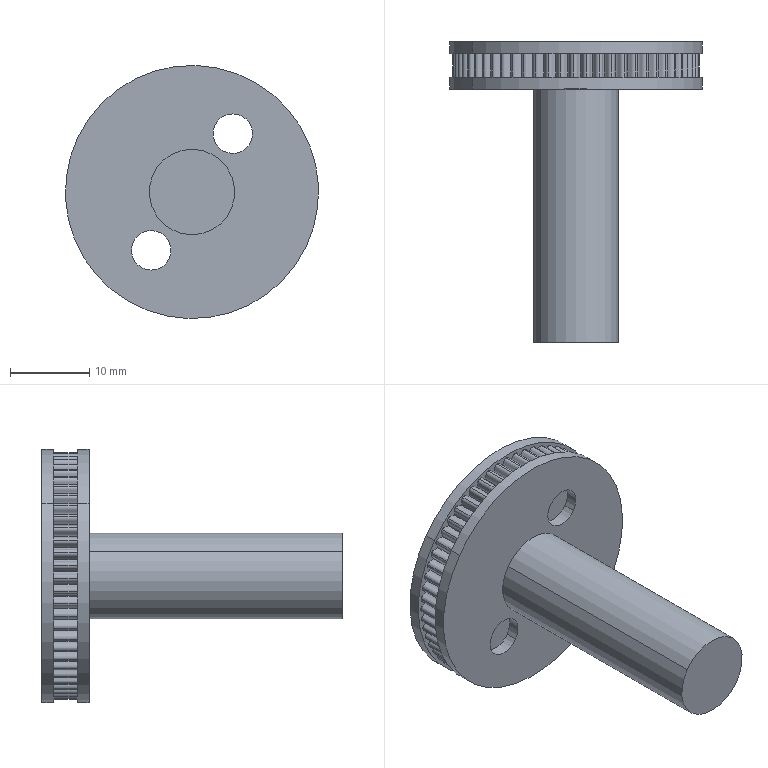Component | SolidWorks | BeltDrive-1 | 1 solid | 143 faces | box 32 x 38 x 32 mm | volume 5637 mm3 | spline 120 | cylinder 16 | plane 7 | commonest cylinder face diameters 5 x8 32 x4 10.8 x2 27.5 x2
build123d program:
from build123d import *

# Parameters (mm, degrees)
SKETCH1_R           = 16
SKETCH1_R_2         = 2.5
BOSS_EXTRUDE1_DEPTH = 1.5
SKETCH2_R           = 14.75
SKETCH2_R_2         = 13.75
BOSS_EXTRUDE2_DEPTH = 3
SKETCH3_R           = 16
SKETCH3_R_2         = 2.5
BOSS_EXTRUDE3_DEPTH = 1.5
SKETCH4_R           = 14.6
BOSS_EXTRUDE4_DEPTH = 3
SKETCH7_R           = 5.4
BOSS_EXTRUDE6_DEPTH = 32


with BuildPart() as part:
    # Sketch1 → Boss-Extrude1 (new body)
    with BuildSketch(Plane.XY):
        Circle(SKETCH1_R)
        with Locations((0, 9)):
            Circle(SKETCH1_R_2, mode=Mode.SUBTRACT)
        with Locations((0, -9)):
            Circle(SKETCH1_R_2, mode=Mode.SUBTRACT)
    extrude(amount=BOSS_EXTRUDE1_DEPTH)

    # Sketch2 → Boss-Extrude2 (add)
    with BuildSketch(Plane.XY.offset(1.5)):
        Circle(SKETCH2_R)
        Circle(SKETCH2_R_2, mode=Mode.SUBTRACT)
    extrude(amount=BOSS_EXTRUDE2_DEPTH)

    # Sketch3 → Boss-Extrude3 (add)
    with BuildSketch(Plane.XY.offset(4.5)):
        Circle(SKETCH3_R)
        with Locations((0, -9)):
            Circle(SKETCH3_R_2, mode=Mode.SUBTRACT)
        with Locations((0, 9)):
            Circle(SKETCH3_R_2, mode=Mode.SUBTRACT)
    extrude(amount=BOSS_EXTRUDE3_DEPTH)

    # Sketch4 → Boss-Extrude4 (add)
    with BuildSketch(Plane.XY.offset(1.5)):
        with BuildLine():
            add(Edge.make_bspline(
                [(0, 15.55), (-0.5399, 15.534), (-0.4124, 15.038), (-0.772, 14.73)],
                knots=[0, 0, 0, 0, 1, 1, 1, 1], degree=3))
            add(Edge.make_bspline(
                [(-1.625, 15.465), (-1.087, 15.505), (-1.162, 14.998), (-0.772, 14.73)],
                knots=[0, 0, 0, 0, 1, 1, 1, 1], degree=3))
            add(Edge.make_bspline(
                [(-1.625, 15.465), (-2.161, 15.392), (-1.982, 14.912), (-2.307, 14.568)],
                knots=[0, 0, 0, 0, 1, 1, 1, 1], degree=3))
            add(Edge.make_bspline(
                [(-3.233, 15.21), (-2.702, 15.307), (-2.723, 14.795), (-2.307, 14.568)],
                knots=[0, 0, 0, 0, 1, 1, 1, 1], degree=3))
            add(Edge.make_bspline(
                [(-3.233, 15.21), (-3.758, 15.082), (-3.53, 14.623), (-3.818, 14.247)],
                knots=[0, 0, 0, 0, 1, 1, 1, 1], degree=3))
            add(Edge.make_bspline(
                [(-4.805, 14.789), (-4.287, 14.94), (-4.255, 14.429), (-3.818, 14.247)],
                knots=[0, 0, 0, 0, 1, 1, 1, 1], degree=3))
            add(Edge.make_bspline(
                [(-4.805, 14.789), (-5.314, 14.607), (-5.039, 14.174), (-5.286, 13.77)],
                knots=[0, 0, 0, 0, 1, 1, 1, 1], degree=3))
            add(Edge.make_bspline(
                [(-6.325, 14.206), (-5.825, 14.41), (-5.74, 13.905), (-5.286, 13.77)],
                knots=[0, 0, 0, 0, 1, 1, 1, 1], degree=3))
            add(Edge.make_bspline(
                [(-6.325, 14.206), (-6.811, 13.971), (-6.493, 13.57), (-6.696, 13.142)],
                knots=[0, 0, 0, 0, 1, 1, 1, 1], degree=3))
            add(Edge.make_bspline(
                [(-7.775, 13.467), (-7.299, 13.723), (-7.162, 13.229), (-6.696, 13.142)],
                knots=[0, 0, 0, 0, 1, 1, 1, 1], degree=3))
            add(Edge.make_bspline(
                [(-7.775, 13.467), (-8.234, 13.183), (-7.876, 12.817), (-8.033, 12.37)],
                knots=[0, 0, 0, 0, 1, 1, 1, 1], degree=3))
            add(Edge.make_bspline(
                [(-9.14, 12.58), (-8.694, 12.884), (-8.505, 12.408), (-8.033, 12.37)],
                knots=[0, 0, 0, 0, 1, 1, 1, 1], degree=3))
            add(Edge.make_bspline(
                [(-9.14, 12.58), (-9.567, 12.25), (-9.173, 11.923), (-9.282, 11.463)],
                knots=[0, 0, 0, 0, 1, 1, 1, 1], degree=3))
            add(Edge.make_bspline(
                [(-10.405, 11.556), (-9.993, 11.905), (-9.756, 11.451), (-9.282, 11.463)],
                knots=[0, 0, 0, 0, 1, 1, 1, 1], degree=3))
            add(Edge.make_bspline(
                [(-10.405, 11.556), (-10.795, 11.183), (-10.369, 10.899), (-10.43, 10.43)],
                knots=[0, 0, 0, 0, 1, 1, 1, 1], degree=3))
            add(Edge.make_bspline(
                [(-11.556, 10.405), (-11.183, 10.795), (-10.899, 10.369), (-10.43, 10.43)],
                knots=[0, 0, 0, 0, 1, 1, 1, 1], degree=3))
            add(Edge.make_bspline(
                [(-11.556, 10.405), (-11.905, 9.993), (-11.451, 9.756), (-11.463, 9.282)],
                knots=[0, 0, 0, 0, 1, 1, 1, 1], degree=3))
            add(Edge.make_bspline(
                [(-12.58, 9.14), (-12.25, 9.567), (-11.923, 9.173), (-11.463, 9.282)],
                knots=[0, 0, 0, 0, 1, 1, 1, 1], degree=3))
            add(Edge.make_bspline(
                [(-12.58, 9.14), (-12.884, 8.694), (-12.408, 8.505), (-12.37, 8.033)],
                knots=[0, 0, 0, 0, 1, 1, 1, 1], degree=3))
            add(Edge.make_bspline(
                [(-13.467, 7.775), (-13.183, 8.234), (-12.817, 7.876), (-12.37, 8.033)],
                knots=[0, 0, 0, 0, 1, 1, 1, 1], degree=3))
            add(Edge.make_bspline(
                [(-13.467, 7.775), (-13.723, 7.299), (-13.229, 7.162), (-13.142, 6.696)],
                knots=[0, 0, 0, 0, 1, 1, 1, 1], degree=3))
            add(Edge.make_bspline(
                [(-14.206, 6.325), (-13.971, 6.811), (-13.57, 6.493), (-13.142, 6.696)],
                knots=[0, 0, 0, 0, 1, 1, 1, 1], degree=3))
            add(Edge.make_bspline(
                [(-14.206, 6.325), (-14.41, 5.825), (-13.905, 5.74), (-13.77, 5.286)],
                knots=[0, 0, 0, 0, 1, 1, 1, 1], degree=3))
            add(Edge.make_bspline(
                [(-14.789, 4.805), (-14.607, 5.314), (-14.174, 5.039), (-13.77, 5.286)],
                knots=[0, 0, 0, 0, 1, 1, 1, 1], degree=3))
            add(Edge.make_bspline(
                [(-14.789, 4.805), (-14.94, 4.287), (-14.429, 4.255), (-14.247, 3.818)],
                knots=[0, 0, 0, 0, 1, 1, 1, 1], degree=3))
            add(Edge.make_bspline(
                [(-15.21, 3.233), (-15.082, 3.758), (-14.623, 3.53), (-14.247, 3.818)],
                knots=[0, 0, 0, 0, 1, 1, 1, 1], degree=3))
            add(Edge.make_bspline(
                [(-15.21, 3.233), (-15.307, 2.702), (-14.795, 2.723), (-14.568, 2.307)],
                knots=[0, 0, 0, 0, 1, 1, 1, 1], degree=3))
            add(Edge.make_bspline(
                [(-15.465, 1.625), (-15.392, 2.161), (-14.912, 1.982), (-14.568, 2.307)],
                knots=[0, 0, 0, 0, 1, 1, 1, 1], degree=3))
            add(Edge.make_bspline(
                [(-15.465, 1.625), (-15.505, 1.087), (-14.998, 1.162), (-14.73, 0.772)],
                knots=[0, 0, 0, 0, 1, 1, 1, 1], degree=3))
            add(Edge.make_bspline(
                [(-15.55, 0), (-15.534, 0.5399), (-15.038, 0.4124), (-14.73, 0.772)],
                knots=[0, 0, 0, 0, 1, 1, 1, 1], degree=3))
            add(Edge.make_bspline(
                [(-15.55, 0), (-15.534, -0.5399), (-15.038, -0.4124), (-14.73, -0.772)],
                knots=[0, 0, 0, 0, 1, 1, 1, 1], degree=3))
            add(Edge.make_bspline(
                [(-15.465, -1.625), (-15.505, -1.087), (-14.998, -1.162), (-14.73, -0.772)],
                knots=[0, 0, 0, 0, 1, 1, 1, 1], degree=3))
            add(Edge.make_bspline(
                [(-15.465, -1.625), (-15.392, -2.161), (-14.912, -1.982), (-14.568, -2.307)],
                knots=[0, 0, 0, 0, 1, 1, 1, 1], degree=3))
            add(Edge.make_bspline(
                [(-15.21, -3.233), (-15.307, -2.702), (-14.795, -2.723), (-14.568, -2.307)],
                knots=[0, 0, 0, 0, 1, 1, 1, 1], degree=3))
            add(Edge.make_bspline(
                [(-15.21, -3.233), (-15.082, -3.758), (-14.623, -3.53), (-14.247, -3.818)],
                knots=[0, 0, 0, 0, 1, 1, 1, 1], degree=3))
            add(Edge.make_bspline(
                [(-14.789, -4.805), (-14.94, -4.287), (-14.429, -4.255), (-14.247, -3.818)],
                knots=[0, 0, 0, 0, 1, 1, 1, 1], degree=3))
            add(Edge.make_bspline(
                [(-14.789, -4.805), (-14.607, -5.314), (-14.174, -5.039), (-13.77, -5.286)],
                knots=[0, 0, 0, 0, 1, 1, 1, 1], degree=3))
            add(Edge.make_bspline(
                [(-14.206, -6.325), (-14.41, -5.825), (-13.905, -5.74), (-13.77, -5.286)],
                knots=[0, 0, 0, 0, 1, 1, 1, 1], degree=3))
            add(Edge.make_bspline(
                [(-14.206, -6.325), (-13.971, -6.811), (-13.57, -6.493), (-13.142, -6.696)],
                knots=[0, 0, 0, 0, 1, 1, 1, 1], degree=3))
            add(Edge.make_bspline(
                [(-13.467, -7.775), (-13.723, -7.299), (-13.229, -7.162), (-13.142, -6.696)],
                knots=[0, 0, 0, 0, 1, 1, 1, 1], degree=3))
            add(Edge.make_bspline(
                [(-13.467, -7.775), (-13.183, -8.234), (-12.817, -7.876), (-12.37, -8.033)],
                knots=[0, 0, 0, 0, 1, 1, 1, 1], degree=3))
            add(Edge.make_bspline(
                [(-12.58, -9.14), (-12.884, -8.694), (-12.408, -8.505), (-12.37, -8.033)],
                knots=[0, 0, 0, 0, 1, 1, 1, 1], degree=3))
            add(Edge.make_bspline(
                [(-12.58, -9.14), (-12.25, -9.567), (-11.923, -9.173), (-11.463, -9.282)],
                knots=[0, 0, 0, 0, 1, 1, 1, 1], degree=3))
            add(Edge.make_bspline(
                [(-11.556, -10.405), (-11.905, -9.993), (-11.451, -9.756), (-11.463, -9.282)],
                knots=[0, 0, 0, 0, 1, 1, 1, 1], degree=3))
            add(Edge.make_bspline(
                [(-11.556, -10.405), (-11.183, -10.795), (-10.899, -10.369), (-10.43, -10.43)],
                knots=[0, 0, 0, 0, 1, 1, 1, 1], degree=3))
            add(Edge.make_bspline(
                [(-10.405, -11.556), (-10.795, -11.183), (-10.369, -10.899), (-10.43, -10.43)],
                knots=[0, 0, 0, 0, 1, 1, 1, 1], degree=3))
            add(Edge.make_bspline(
                [(-10.405, -11.556), (-9.993, -11.905), (-9.756, -11.451), (-9.282, -11.463)],
                knots=[0, 0, 0, 0, 1, 1, 1, 1], degree=3))
            add(Edge.make_bspline(
                [(-9.14, -12.58), (-9.567, -12.25), (-9.173, -11.923), (-9.282, -11.463)],
                knots=[0, 0, 0, 0, 1, 1, 1, 1], degree=3))
            add(Edge.make_bspline(
                [(-9.14, -12.58), (-8.694, -12.884), (-8.505, -12.408), (-8.033, -12.37)],
                knots=[0, 0, 0, 0, 1, 1, 1, 1], degree=3))
            add(Edge.make_bspline(
                [(-7.775, -13.467), (-8.234, -13.183), (-7.876, -12.817), (-8.033, -12.37)],
                knots=[0, 0, 0, 0, 1, 1, 1, 1], degree=3))
            add(Edge.make_bspline(
                [(-7.775, -13.467), (-7.299, -13.723), (-7.162, -13.229), (-6.696, -13.142)],
                knots=[0, 0, 0, 0, 1, 1, 1, 1], degree=3))
            add(Edge.make_bspline(
                [(-6.325, -14.206), (-6.811, -13.971), (-6.493, -13.57), (-6.696, -13.142)],
                knots=[0, 0, 0, 0, 1, 1, 1, 1], degree=3))
            add(Edge.make_bspline(
                [(-6.325, -14.206), (-5.825, -14.41), (-5.74, -13.905), (-5.286, -13.77)],
                knots=[0, 0, 0, 0, 1, 1, 1, 1], degree=3))
            add(Edge.make_bspline(
                [(-4.805, -14.789), (-5.314, -14.607), (-5.039, -14.174), (-5.286, -13.77)],
                knots=[0, 0, 0, 0, 1, 1, 1, 1], degree=3))
            add(Edge.make_bspline(
                [(-4.805, -14.789), (-4.287, -14.94), (-4.255, -14.429), (-3.818, -14.247)],
                knots=[0, 0, 0, 0, 1, 1, 1, 1], degree=3))
            add(Edge.make_bspline(
                [(-3.233, -15.21), (-3.758, -15.082), (-3.53, -14.623), (-3.818, -14.247)],
                knots=[0, 0, 0, 0, 1, 1, 1, 1], degree=3))
            add(Edge.make_bspline(
                [(-3.233, -15.21), (-2.702, -15.307), (-2.723, -14.795), (-2.307, -14.568)],
                knots=[0, 0, 0, 0, 1, 1, 1, 1], degree=3))
            add(Edge.make_bspline(
                [(-1.625, -15.465), (-2.161, -15.392), (-1.982, -14.912), (-2.307, -14.568)],
                knots=[0, 0, 0, 0, 1, 1, 1, 1], degree=3))
            add(Edge.make_bspline(
                [(-1.625, -15.465), (-1.087, -15.505), (-1.162, -14.998), (-0.772, -14.73)],
                knots=[0, 0, 0, 0, 1, 1, 1, 1], degree=3))
            add(Edge.make_bspline(
                [(0, -15.55), (-0.5399, -15.534), (-0.4124, -15.038), (-0.772, -14.73)],
                knots=[0, 0, 0, 0, 1, 1, 1, 1], degree=3))
            add(Edge.make_bspline(
                [(0, -15.55), (0.5399, -15.534), (0.4124, -15.038), (0.772, -14.73)],
                knots=[0, 0, 0, 0, 1, 1, 1, 1], degree=3))
            add(Edge.make_bspline(
                [(1.625, -15.465), (1.087, -15.505), (1.162, -14.998), (0.772, -14.73)],
                knots=[0, 0, 0, 0, 1, 1, 1, 1], degree=3))
            add(Edge.make_bspline(
                [(1.625, -15.465), (2.161, -15.392), (1.982, -14.912), (2.307, -14.568)],
                knots=[0, 0, 0, 0, 1, 1, 1, 1], degree=3))
            add(Edge.make_bspline(
                [(3.233, -15.21), (2.702, -15.307), (2.723, -14.795), (2.307, -14.568)],
                knots=[0, 0, 0, 0, 1, 1, 1, 1], degree=3))
            add(Edge.make_bspline(
                [(3.233, -15.21), (3.758, -15.082), (3.53, -14.623), (3.818, -14.247)],
                knots=[0, 0, 0, 0, 1, 1, 1, 1], degree=3))
            add(Edge.make_bspline(
                [(4.805, -14.789), (4.287, -14.94), (4.255, -14.429), (3.818, -14.247)],
                knots=[0, 0, 0, 0, 1, 1, 1, 1], degree=3))
            add(Edge.make_bspline(
                [(4.805, -14.789), (5.314, -14.607), (5.039, -14.174), (5.286, -13.77)],
                knots=[0, 0, 0, 0, 1, 1, 1, 1], degree=3))
            add(Edge.make_bspline(
                [(6.325, -14.206), (5.825, -14.41), (5.74, -13.905), (5.286, -13.77)],
                knots=[0, 0, 0, 0, 1, 1, 1, 1], degree=3))
            add(Edge.make_bspline(
                [(6.325, -14.206), (6.811, -13.971), (6.493, -13.57), (6.696, -13.142)],
                knots=[0, 0, 0, 0, 1, 1, 1, 1], degree=3))
            add(Edge.make_bspline(
                [(7.775, -13.467), (7.299, -13.723), (7.162, -13.229), (6.696, -13.142)],
                knots=[0, 0, 0, 0, 1, 1, 1, 1], degree=3))
            add(Edge.make_bspline(
                [(7.775, -13.467), (8.234, -13.183), (7.876, -12.817), (8.033, -12.37)],
                knots=[0, 0, 0, 0, 1, 1, 1, 1], degree=3))
            add(Edge.make_bspline(
                [(9.14, -12.58), (8.694, -12.884), (8.505, -12.408), (8.033, -12.37)],
                knots=[0, 0, 0, 0, 1, 1, 1, 1], degree=3))
            add(Edge.make_bspline(
                [(9.14, -12.58), (9.567, -12.25), (9.173, -11.923), (9.282, -11.463)],
                knots=[0, 0, 0, 0, 1, 1, 1, 1], degree=3))
            add(Edge.make_bspline(
                [(10.405, -11.556), (9.993, -11.905), (9.756, -11.451), (9.282, -11.463)],
                knots=[0, 0, 0, 0, 1, 1, 1, 1], degree=3))
            add(Edge.make_bspline(
                [(10.405, -11.556), (10.795, -11.183), (10.369, -10.899), (10.43, -10.43)],
                knots=[0, 0, 0, 0, 1, 1, 1, 1], degree=3))
            add(Edge.make_bspline(
                [(11.556, -10.405), (11.183, -10.795), (10.899, -10.369), (10.43, -10.43)],
                knots=[0, 0, 0, 0, 1, 1, 1, 1], degree=3))
            add(Edge.make_bspline(
                [(11.556, -10.405), (11.905, -9.993), (11.451, -9.756), (11.463, -9.282)],
                knots=[0, 0, 0, 0, 1, 1, 1, 1], degree=3))
            add(Edge.make_bspline(
                [(12.58, -9.14), (12.25, -9.567), (11.923, -9.173), (11.463, -9.282)],
                knots=[0, 0, 0, 0, 1, 1, 1, 1], degree=3))
            add(Edge.make_bspline(
                [(12.58, -9.14), (12.884, -8.694), (12.408, -8.505), (12.37, -8.033)],
                knots=[0, 0, 0, 0, 1, 1, 1, 1], degree=3))
            add(Edge.make_bspline(
                [(13.467, -7.775), (13.183, -8.234), (12.817, -7.876), (12.37, -8.033)],
                knots=[0, 0, 0, 0, 1, 1, 1, 1], degree=3))
            add(Edge.make_bspline(
                [(13.467, -7.775), (13.723, -7.299), (13.229, -7.162), (13.142, -6.696)],
                knots=[0, 0, 0, 0, 1, 1, 1, 1], degree=3))
            add(Edge.make_bspline(
                [(14.206, -6.325), (13.971, -6.811), (13.57, -6.493), (13.142, -6.696)],
                knots=[0, 0, 0, 0, 1, 1, 1, 1], degree=3))
            add(Edge.make_bspline(
                [(14.206, -6.325), (14.41, -5.825), (13.905, -5.74), (13.77, -5.286)],
                knots=[0, 0, 0, 0, 1, 1, 1, 1], degree=3))
            add(Edge.make_bspline(
                [(14.789, -4.805), (14.607, -5.314), (14.174, -5.039), (13.77, -5.286)],
                knots=[0, 0, 0, 0, 1, 1, 1, 1], degree=3))
            add(Edge.make_bspline(
                [(14.789, -4.805), (14.94, -4.287), (14.429, -4.255), (14.247, -3.818)],
                knots=[0, 0, 0, 0, 1, 1, 1, 1], degree=3))
            add(Edge.make_bspline(
                [(15.21, -3.233), (15.082, -3.758), (14.623, -3.53), (14.247, -3.818)],
                knots=[0, 0, 0, 0, 1, 1, 1, 1], degree=3))
            add(Edge.make_bspline(
                [(15.21, -3.233), (15.307, -2.702), (14.795, -2.723), (14.568, -2.307)],
                knots=[0, 0, 0, 0, 1, 1, 1, 1], degree=3))
            add(Edge.make_bspline(
                [(15.465, -1.625), (15.392, -2.161), (14.912, -1.982), (14.568, -2.307)],
                knots=[0, 0, 0, 0, 1, 1, 1, 1], degree=3))
            add(Edge.make_bspline(
                [(15.465, -1.625), (15.505, -1.087), (14.998, -1.162), (14.73, -0.772)],
                knots=[0, 0, 0, 0, 1, 1, 1, 1], degree=3))
            add(Edge.make_bspline(
                [(15.55, 0), (15.534, -0.5399), (15.038, -0.4124), (14.73, -0.772)],
                knots=[0, 0, 0, 0, 1, 1, 1, 1], degree=3))
            add(Edge.make_bspline(
                [(15.55, 0), (15.534, 0.5399), (15.038, 0.4124), (14.73, 0.772)],
                knots=[0, 0, 0, 0, 1, 1, 1, 1], degree=3))
            add(Edge.make_bspline(
                [(15.465, 1.625), (15.505, 1.087), (14.998, 1.162), (14.73, 0.772)],
                knots=[0, 0, 0, 0, 1, 1, 1, 1], degree=3))
            add(Edge.make_bspline(
                [(15.465, 1.625), (15.392, 2.161), (14.912, 1.982), (14.568, 2.307)],
                knots=[0, 0, 0, 0, 1, 1, 1, 1], degree=3))
            add(Edge.make_bspline(
                [(15.21, 3.233), (15.307, 2.702), (14.795, 2.723), (14.568, 2.307)],
                knots=[0, 0, 0, 0, 1, 1, 1, 1], degree=3))
            add(Edge.make_bspline(
                [(15.21, 3.233), (15.082, 3.758), (14.623, 3.53), (14.247, 3.818)],
                knots=[0, 0, 0, 0, 1, 1, 1, 1], degree=3))
            add(Edge.make_bspline(
                [(14.789, 4.805), (14.94, 4.287), (14.429, 4.255), (14.247, 3.818)],
                knots=[0, 0, 0, 0, 1, 1, 1, 1], degree=3))
            add(Edge.make_bspline(
                [(14.789, 4.805), (14.607, 5.314), (14.174, 5.039), (13.77, 5.286)],
                knots=[0, 0, 0, 0, 1, 1, 1, 1], degree=3))
            add(Edge.make_bspline(
                [(14.206, 6.325), (14.41, 5.825), (13.905, 5.74), (13.77, 5.286)],
                knots=[0, 0, 0, 0, 1, 1, 1, 1], degree=3))
            add(Edge.make_bspline(
                [(14.206, 6.325), (13.971, 6.811), (13.57, 6.493), (13.142, 6.696)],
                knots=[0, 0, 0, 0, 1, 1, 1, 1], degree=3))
            add(Edge.make_bspline(
                [(13.467, 7.775), (13.723, 7.299), (13.229, 7.162), (13.142, 6.696)],
                knots=[0, 0, 0, 0, 1, 1, 1, 1], degree=3))
            add(Edge.make_bspline(
                [(13.467, 7.775), (13.183, 8.234), (12.817, 7.876), (12.37, 8.033)],
                knots=[0, 0, 0, 0, 1, 1, 1, 1], degree=3))
            add(Edge.make_bspline(
                [(12.58, 9.14), (12.884, 8.694), (12.408, 8.505), (12.37, 8.033)],
                knots=[0, 0, 0, 0, 1, 1, 1, 1], degree=3))
            add(Edge.make_bspline(
                [(12.58, 9.14), (12.25, 9.567), (11.923, 9.173), (11.463, 9.282)],
                knots=[0, 0, 0, 0, 1, 1, 1, 1], degree=3))
            add(Edge.make_bspline(
                [(11.556, 10.405), (11.905, 9.993), (11.451, 9.756), (11.463, 9.282)],
                knots=[0, 0, 0, 0, 1, 1, 1, 1], degree=3))
            add(Edge.make_bspline(
                [(11.556, 10.405), (11.183, 10.795), (10.899, 10.369), (10.43, 10.43)],
                knots=[0, 0, 0, 0, 1, 1, 1, 1], degree=3))
            add(Edge.make_bspline(
                [(10.405, 11.556), (10.795, 11.183), (10.369, 10.899), (10.43, 10.43)],
                knots=[0, 0, 0, 0, 1, 1, 1, 1], degree=3))
            add(Edge.make_bspline(
                [(10.405, 11.556), (9.993, 11.905), (9.756, 11.451), (9.282, 11.463)],
                knots=[0, 0, 0, 0, 1, 1, 1, 1], degree=3))
            add(Edge.make_bspline(
                [(9.14, 12.58), (9.567, 12.25), (9.173, 11.923), (9.282, 11.463)],
                knots=[0, 0, 0, 0, 1, 1, 1, 1], degree=3))
            add(Edge.make_bspline(
                [(9.14, 12.58), (8.694, 12.884), (8.505, 12.408), (8.033, 12.37)],
                knots=[0, 0, 0, 0, 1, 1, 1, 1], degree=3))
            add(Edge.make_bspline(
                [(7.775, 13.467), (8.234, 13.183), (7.876, 12.817), (8.033, 12.37)],
                knots=[0, 0, 0, 0, 1, 1, 1, 1], degree=3))
            add(Edge.make_bspline(
                [(7.775, 13.467), (7.299, 13.723), (7.162, 13.229), (6.696, 13.142)],
                knots=[0, 0, 0, 0, 1, 1, 1, 1], degree=3))
            add(Edge.make_bspline(
                [(6.325, 14.206), (6.811, 13.971), (6.493, 13.57), (6.696, 13.142)],
                knots=[0, 0, 0, 0, 1, 1, 1, 1], degree=3))
            add(Edge.make_bspline(
                [(6.325, 14.206), (5.825, 14.41), (5.74, 13.905), (5.286, 13.77)],
                knots=[0, 0, 0, 0, 1, 1, 1, 1], degree=3))
            add(Edge.make_bspline(
                [(4.805, 14.789), (5.314, 14.607), (5.039, 14.174), (5.286, 13.77)],
                knots=[0, 0, 0, 0, 1, 1, 1, 1], degree=3))
            add(Edge.make_bspline(
                [(4.805, 14.789), (4.287, 14.94), (4.255, 14.429), (3.818, 14.247)],
                knots=[0, 0, 0, 0, 1, 1, 1, 1], degree=3))
            add(Edge.make_bspline(
                [(3.233, 15.21), (3.758, 15.082), (3.53, 14.623), (3.818, 14.247)],
                knots=[0, 0, 0, 0, 1, 1, 1, 1], degree=3))
            add(Edge.make_bspline(
                [(3.233, 15.21), (2.702, 15.307), (2.723, 14.795), (2.307, 14.568)],
                knots=[0, 0, 0, 0, 1, 1, 1, 1], degree=3))
            add(Edge.make_bspline(
                [(1.625, 15.465), (2.161, 15.392), (1.982, 14.912), (2.307, 14.568)],
                knots=[0, 0, 0, 0, 1, 1, 1, 1], degree=3))
            add(Edge.make_bspline(
                [(1.625, 15.465), (1.087, 15.505), (1.162, 14.998), (0.772, 14.73)],
                knots=[0, 0, 0, 0, 1, 1, 1, 1], degree=3))
            add(Edge.make_bspline(
                [(0, 15.55), (0.5399, 15.534), (0.4124, 15.038), (0.772, 14.73)],
                knots=[0, 0, 0, 0, 1, 1, 1, 1], degree=3))
        make_face()
        Circle(SKETCH4_R, mode=Mode.SUBTRACT)
    extrude(amount=BOSS_EXTRUDE4_DEPTH)

    # Sketch7 → Boss-Extrude6 (add)
    with BuildSketch(Plane(origin=(0, 0, 0), x_dir=(-1, 0, 0), z_dir=(0, 0, -1))):
        Circle(SKETCH7_R)
    extrude(amount=BOSS_EXTRUDE6_DEPTH)


solid = part.part

# Placed as in the assembly
solid = solid.moved(Location((-102.554, 516.247, 900.064), (-90, 0, -145.024)))